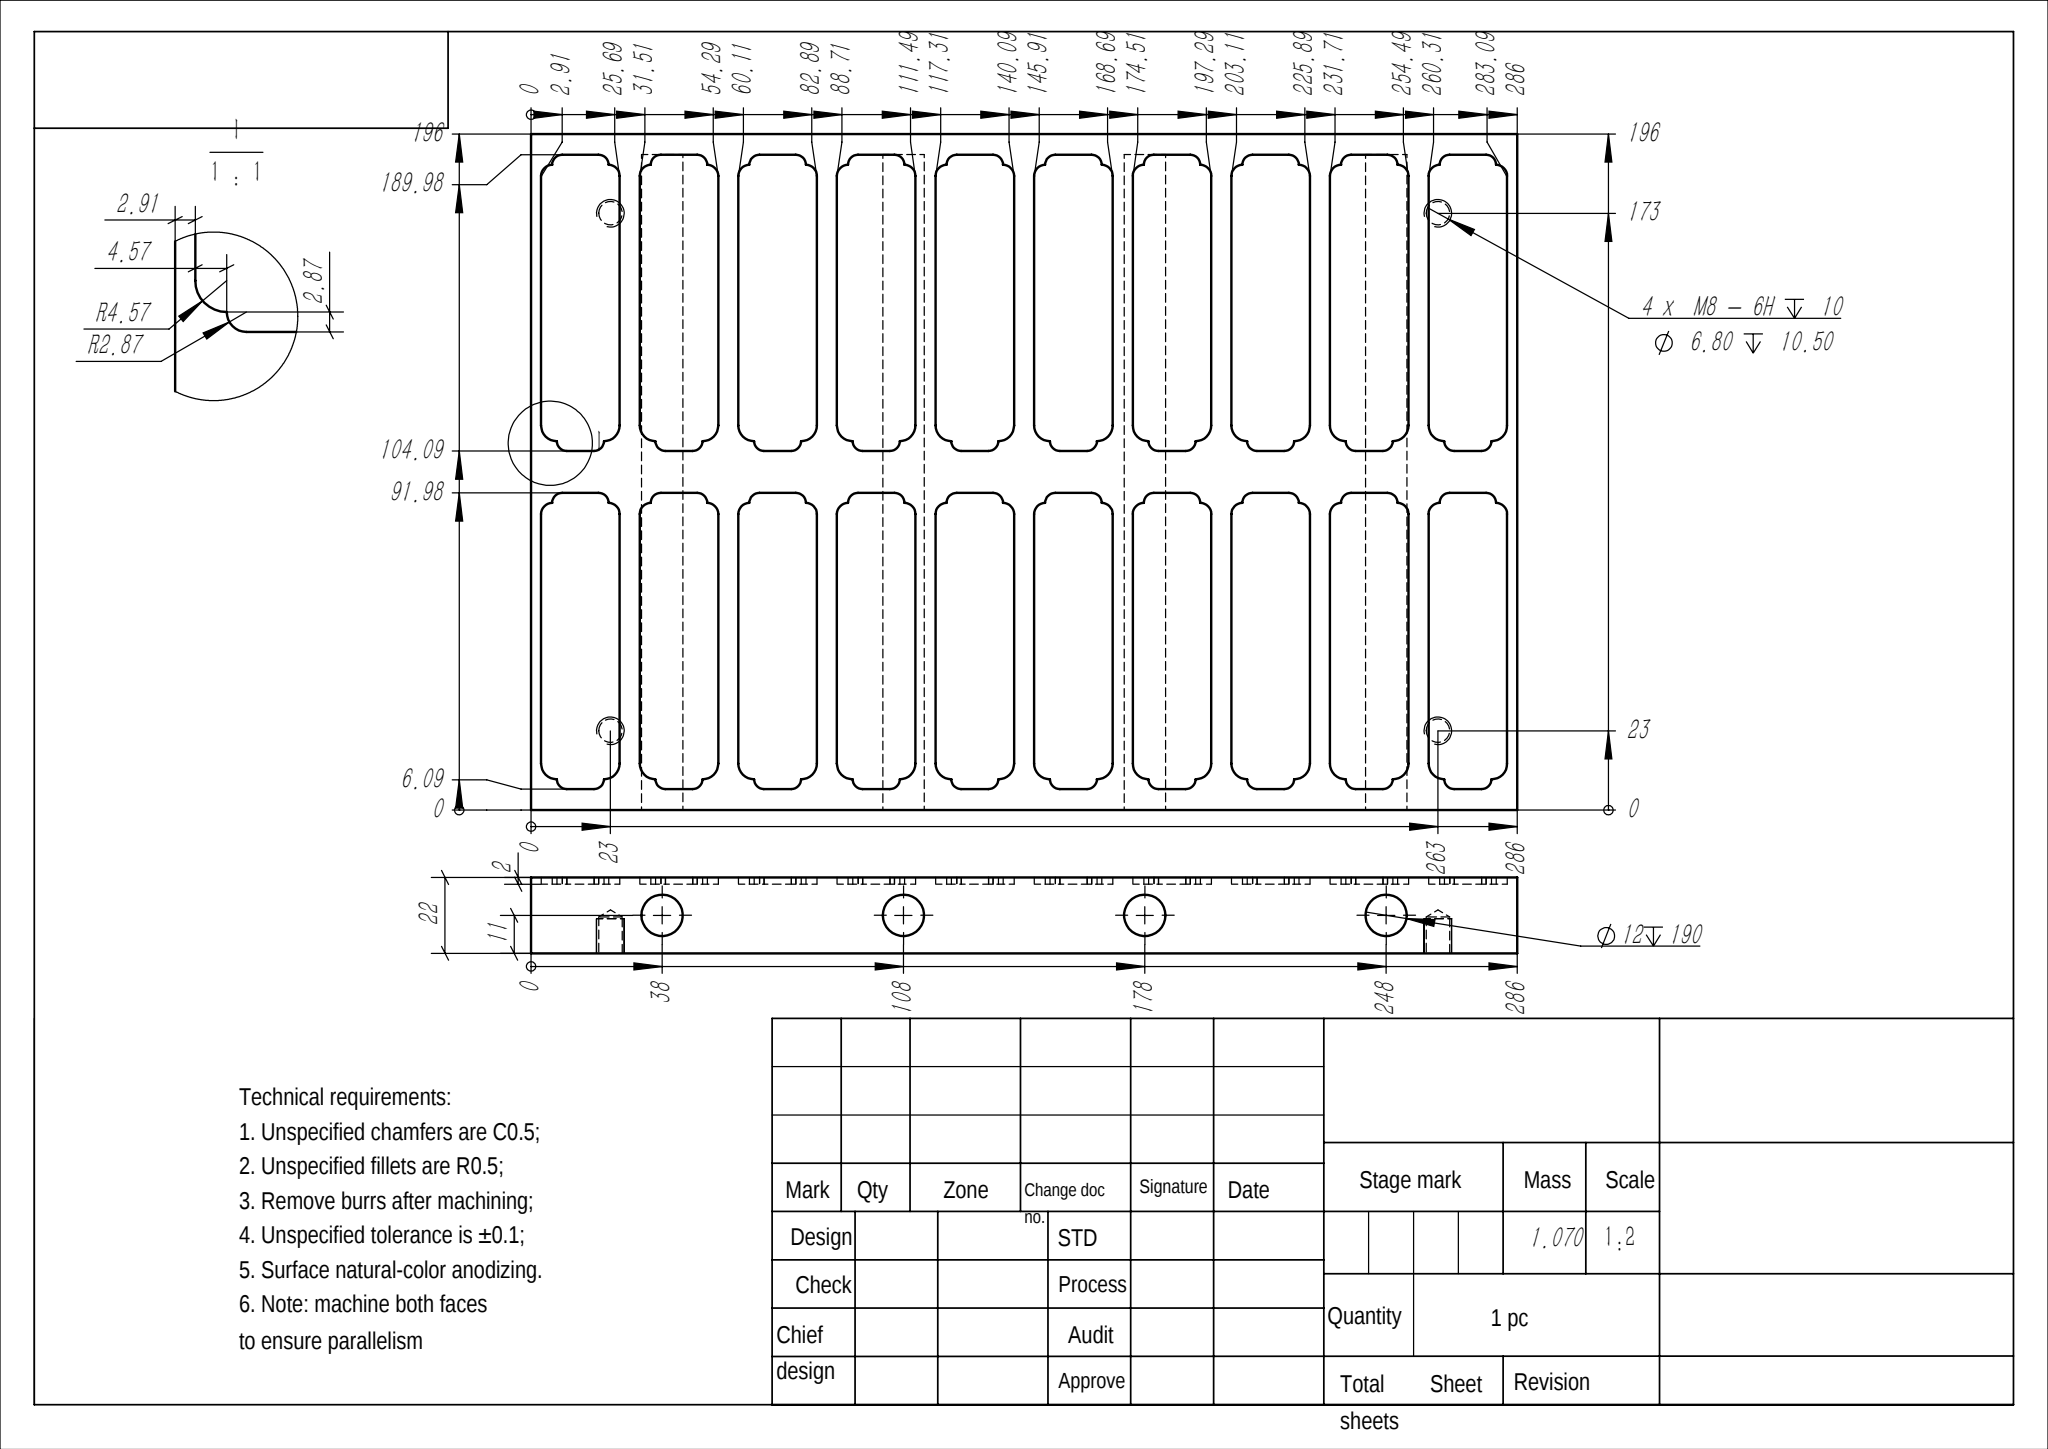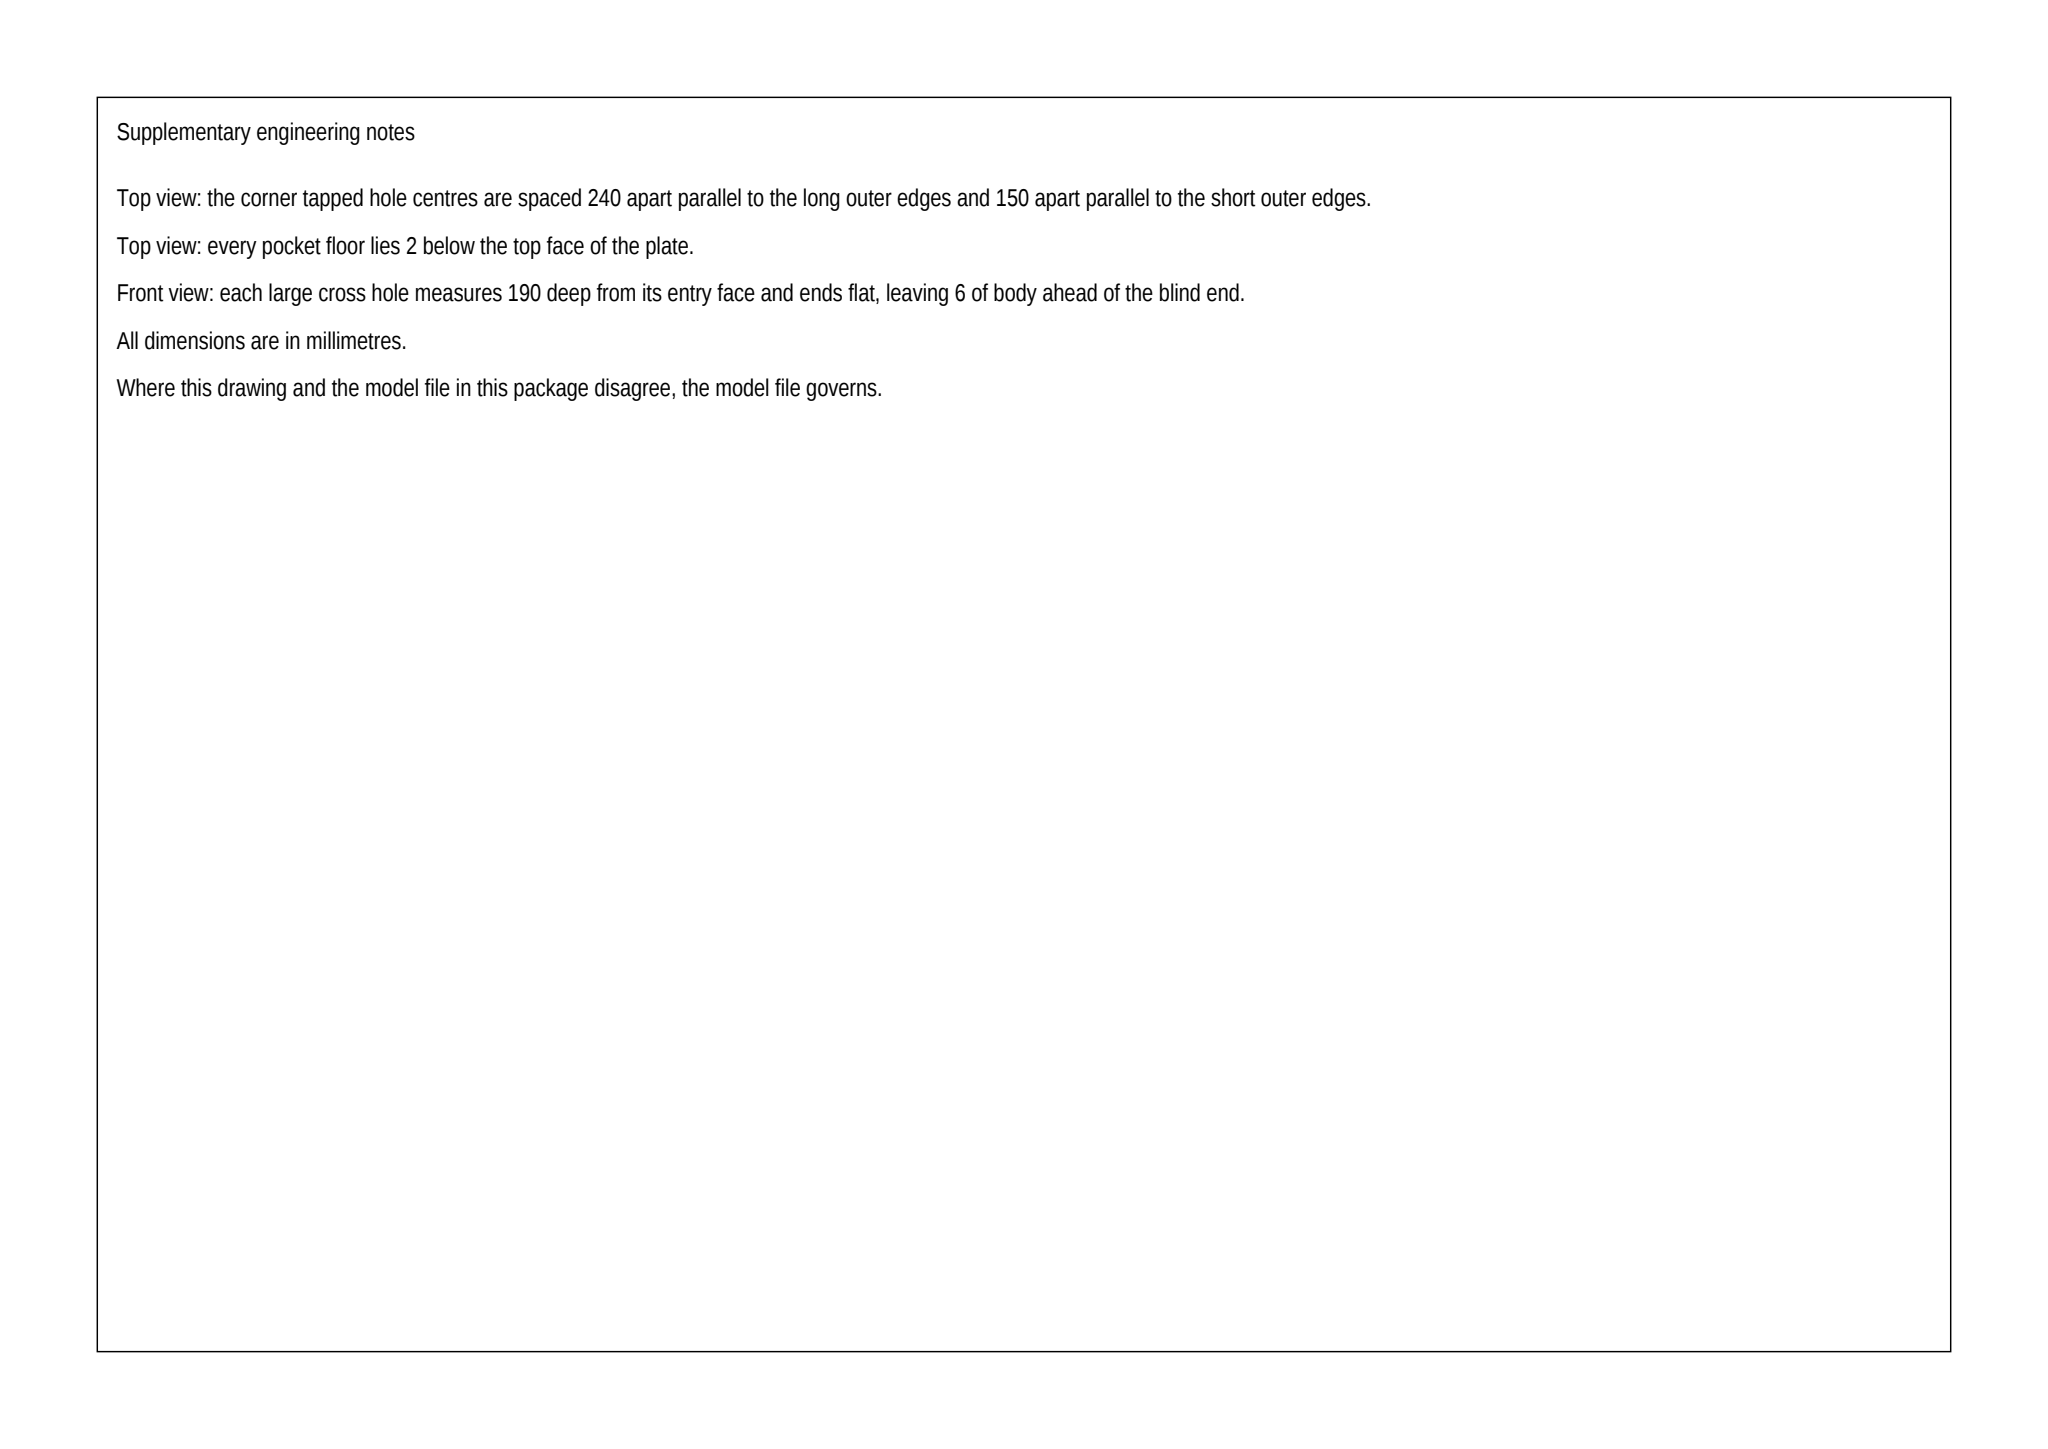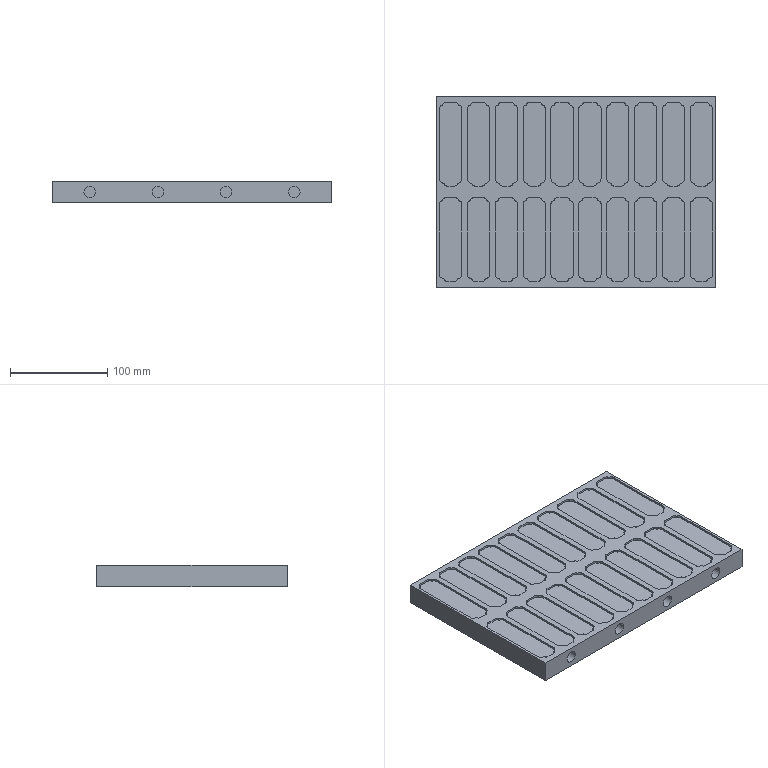Part | SolidWorks | mm | 1 solid | 294 faces | box 286 x 196 x 22 mm | volume 1070011 mm3 | cylinder 176 | plane 110 | cone 8 | commonest cylinder face diameters 5.86 x40 6.4 x40 5.74 x40 9.14 x40 12 x8 6.8 x8